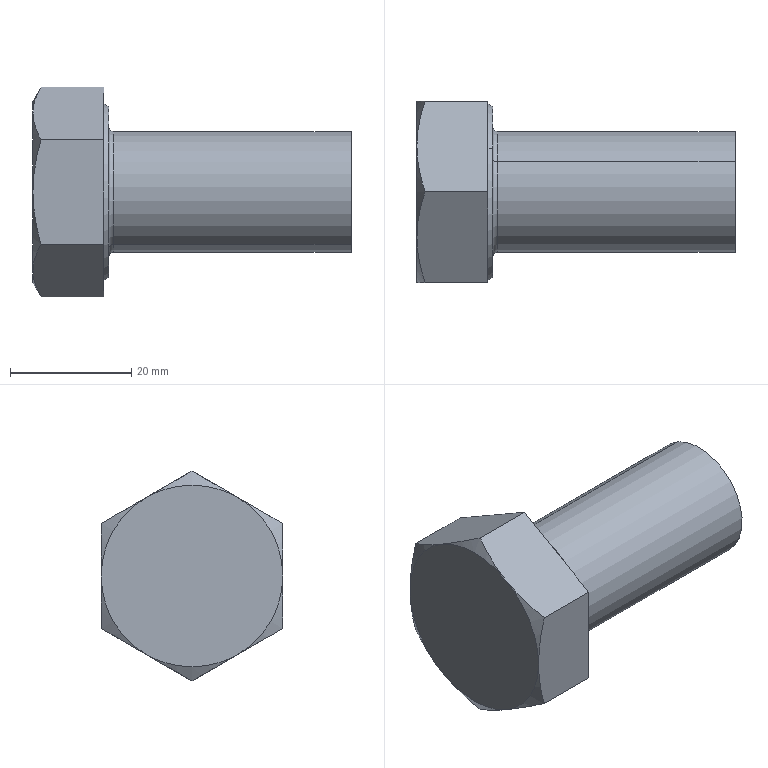Component | SolidWorks | GB_T5782-2016[HexHeadBoltM20_40]-1 | 1 solid | 22 faces | box 52.5 x 30 x 34.64 mm | volume 22181 mm3 | plane 10 | cone 8 | torus 2 | cylinder 2 | commonest cylinder face diameters 20 x2
build123d program:
from build123d import *

# Parameters (mm, degrees)
BASE_EXTRUDE_DEPTH = 12.5
FILLET_2_R         = 0.8
MOVE_FACE1_BY      = 40


with BuildPart() as part:
    # Sketch1 → Base-Extrude (new body)
    with BuildSketch(Plane(origin=(0, 0, 0), x_dir=(0, 0, -1), z_dir=(1, 0, 0))):
        Polygon((15, 8.66), (15, -8.66), (0, -17.321), (-15, -8.66), (-15, 8.66), (0, 17.321), align=None)
    extrude(amount=BASE_EXTRUDE_DEPTH)

    # Sketch2 → Revolve1 (revolve)
    with BuildSketch(Plane.XY, mode=Mode.PRIVATE) as revolve1_sk:
        Polygon((0, 0), (92.5, 0), (92.5, 7.835), (92.5, 10), (46.5, 10), (0, 10), align=None)
    revolve(revolve1_sk.sketch.rotate(Axis((0, 0, 0), (1, 0, 0)), 90), axis=Axis((0, 0, 0), (1, 0, 0)))

    # Sketch3 → Cut-Revolve1 (revolve, cut)
    with BuildSketch(Plane.XY):
        Polygon((0, 15), (4.226, 22.321), (4.226, 27.321), (-10, 27.321), (-10, 15), align=None)
    revolve(axis=Axis((0, 0, 0), (1, 0, 0)), mode=Mode.SUBTRACT)

    # Sketch4 → Cut-Revolve3 (revolve, cut)
    with BuildSketch(Plane.XY, mode=Mode.PRIVATE) as cut_revolve3_sk:
        Polygon((12.5, 14.095), (11.7, 14.557), (11.7, 17.321), (12.5, 17.321), align=None)
    revolve(cut_revolve3_sk.sketch.rotate(Axis((0, 0, 0), (1, 0, 0)), 90), axis=Axis((0, 0, 0), (1, 0, 0)), mode=Mode.SUBTRACT)

    # Fillet 2
    fillet_2_edges = [part.edges().sort_by_distance(p)[0] for p in [
        (12.5, 0, -10),
    ]]
    fillet(fillet_2_edges, radius=FILLET_2_R)

    # Move Face1: a face moved inward by 40.0
    extrude(part.faces().sort_by_distance((92.5, 0, 0))[0], amount=MOVE_FACE1_BY, dir=(-1, 0, 0), mode=Mode.SUBTRACT)


solid = part.part

# Placed as in the assembly
solid = solid.moved(Location((-212, -402, 70), (90, 0, 0)))
STEP:
#1=CARTESIAN_POINT('',(-7.823,-15.63,3.097));
#2=VERTEX_POINT('',#1);
#3=CARTESIAN_POINT('',(-7.823,-16.024,2.415));
#4=VERTEX_POINT('',#3);
#5=CARTESIAN_POINT('',(-7.823,-15.827,2.756));
#6=DIRECTION('',(1.,0.,0.));
#7=DIRECTION('',(0.,-0.5,-0.866));
#8=AXIS2_PLACEMENT_3D('',#5,#6,#7);
#9=CIRCLE('',#8,0.3937);
#10=EDGE_CURVE('',#2,#4,#9,.T.);
#11=ORIENTED_EDGE('',*,*,#10,.F.);
#12=CARTESIAN_POINT('',(-7.854,-15.614,3.124));
#13=VERTEX_POINT('',#12);
#14=CARTESIAN_POINT('',(-7.823,-15.614,3.124));
#15=DIRECTION('',(0.,0.866,-0.5));
#16=DIRECTION('',(0.,0.5,0.866));
#17=AXIS2_PLACEMENT_3D('',#14,#15,#16);
#18=CIRCLE('',#17,0.0315);
#19=EDGE_CURVE('',#2,#13,#18,.T.);
#20=ORIENTED_EDGE('',*,*,#19,.T.);
#21=CARTESIAN_POINT('',(-7.854,-16.039,2.388));
#22=VERTEX_POINT('',#21);
#23=CARTESIAN_POINT('',(-7.854,-15.827,2.756));
#24=DIRECTION('',(-1.,0.,0.));
#25=DIRECTION('',(0.,-0.5,-0.866));
#26=AXIS2_PLACEMENT_3D('',#23,#24,#25);
#27=CIRCLE('',#26,0.4252);
#28=EDGE_CURVE('',#22,#13,#27,.T.);
#29=ORIENTED_EDGE('',*,*,#28,.F.);
#30=CARTESIAN_POINT('',(-7.823,-16.039,2.388));
#31=DIRECTION('',(0.,-0.866,0.5));
#32=DIRECTION('',(0.,-0.5,-0.866));
#33=AXIS2_PLACEMENT_3D('',#30,#31,#32);
#34=CIRCLE('',#33,0.0315);
#35=EDGE_CURVE('',#4,#22,#34,.T.);
#36=ORIENTED_EDGE('',*,*,#35,.F.);
#37=EDGE_LOOP('',(#11,#20,#29,#36));
#38=FACE_OUTER_BOUND('',#37,.T.);
#39=CARTESIAN_POINT('',(-7.823,-15.827,2.756));
#40=DIRECTION('',(1.,0.,0.));
#41=DIRECTION('',(0.,-0.5,-0.866));
#42=AXIS2_PLACEMENT_3D('',#39,#40,#41);
#43=TOROIDAL_SURFACE('',#42,0.4252,0.0315);
#44=ADVANCED_FACE('',(#38),#43,.F.);
#45=CARTESIAN_POINT('',(-6.28,-15.63,3.097));
#46=VERTEX_POINT('',#45);
#47=CARTESIAN_POINT('',(-6.28,-16.024,2.415));
#48=VERTEX_POINT('',#47);
#49=CARTESIAN_POINT('',(-6.28,-15.827,2.756));
#50=DIRECTION('',(-1.,0.,0.));
#51=DIRECTION('',(0.,0.5,0.866));
#52=AXIS2_PLACEMENT_3D('',#49,#50,#51);
#53=CIRCLE('',#52,0.3937);
#54=EDGE_CURVE('',#46,#48,#53,.T.);
#55=ORIENTED_EDGE('',*,*,#54,.T.);
#56=CARTESIAN_POINT('',(-8.346,-16.024,2.415));
#57=DIRECTION('',(-1.,0.,0.));
#58=VECTOR('',#57,39.37);
#59=LINE('',#56,#58);
#60=EDGE_CURVE('',#48,#4,#59,.T.);
#61=ORIENTED_EDGE('',*,*,#60,.T.);
#62=CARTESIAN_POINT('',(-7.823,-15.827,2.756));
#63=DIRECTION('',(1.,0.,0.));
#64=DIRECTION('',(0.,-0.5,-0.866));
#65=AXIS2_PLACEMENT_3D('',#62,#63,#64);
#66=CIRCLE('',#65,0.3937);
#67=EDGE_CURVE('',#4,#2,#66,.T.);
#68=ORIENTED_EDGE('',*,*,#67,.T.);
#69=CARTESIAN_POINT('',(-8.346,-15.63,3.097));
#70=DIRECTION('',(-1.,0.,0.));
#71=VECTOR('',#70,39.37);
#72=LINE('',#69,#71);
#73=EDGE_CURVE('',#46,#2,#72,.T.);
#74=ORIENTED_EDGE('',*,*,#73,.F.);
#75=EDGE_LOOP('',(#55,#61,#68,#74));
#76=FACE_OUTER_BOUND('',#75,.T.);
#77=CARTESIAN_POINT('',(-8.346,-15.827,2.756));
#78=DIRECTION('',(-1.,0.,0.));
#79=DIRECTION('',(0.,0.5,0.866));
#80=AXIS2_PLACEMENT_3D('',#77,#78,#79);
#81=CYLINDRICAL_SURFACE('',#80,0.3937);
#82=ADVANCED_FACE('',(#76),#81,.T.);
#83=CARTESIAN_POINT('',(-7.854,-15.549,3.236));
#84=VERTEX_POINT('',#83);
#85=CARTESIAN_POINT('',(-7.854,-16.104,2.275));
#86=VERTEX_POINT('',#85);
#87=CARTESIAN_POINT('',(-7.854,-15.827,2.756));
#88=DIRECTION('',(-1.,0.,0.));
#89=DIRECTION('',(0.,0.5,0.866));
#90=AXIS2_PLACEMENT_3D('',#87,#88,#89);
#91=CIRCLE('',#90,0.5549);
#92=EDGE_CURVE('',#84,#86,#91,.T.);
#93=ORIENTED_EDGE('',*,*,#92,.T.);
#94=CARTESIAN_POINT('',(-7.886,-16.113,2.26));
#95=VERTEX_POINT('',#94);
#96=CARTESIAN_POINT('',(-7.886,-16.113,2.26));
#97=DIRECTION('',(-0.866,-0.25,-0.433));
#98=VECTOR('',#97,39.37);
#99=LINE('',#96,#98);
#100=EDGE_CURVE('',#86,#95,#99,.T.);
#101=ORIENTED_EDGE('',*,*,#100,.T.);
#102=CARTESIAN_POINT('',(-7.886,-15.54,3.252));
#103=VERTEX_POINT('',#102);
#104=CARTESIAN_POINT('',(-7.886,-15.827,2.756));
#105=DIRECTION('',(-1.,0.,0.));
#106=DIRECTION('',(0.,0.5,0.866));
#107=AXIS2_PLACEMENT_3D('',#104,#105,#106);
#108=CIRCLE('',#107,0.5731);
#109=EDGE_CURVE('',#103,#95,#108,.T.);
#110=ORIENTED_EDGE('',*,*,#109,.F.);
#111=CARTESIAN_POINT('',(-7.886,-15.54,3.252));
#112=DIRECTION('',(-0.866,0.25,0.433));
#113=VECTOR('',#112,39.37);
#114=LINE('',#111,#113);
#115=EDGE_CURVE('',#84,#103,#114,.T.);
#116=ORIENTED_EDGE('',*,*,#115,.F.);
#117=EDGE_LOOP('',(#93,#101,#110,#116));
#118=FACE_OUTER_BOUND('',#117,.T.);
#119=CARTESIAN_POINT('',(-7.886,-15.827,2.756));
#120=DIRECTION('',(-1.,0.,0.));
#121=DIRECTION('',(0.,0.5,0.866));
#122=AXIS2_PLACEMENT_3D('',#119,#120,#121);
#123=CONICAL_SURFACE('',#122,0.5731,0.5236);
#124=ADVANCED_FACE('',(#118),#123,.T.);
#125=CARTESIAN_POINT('',(-7.886,-15.827,2.074));
#126=VERTEX_POINT('',#125);
#127=CARTESIAN_POINT('',(-7.886,-15.236,2.415));
#128=VERTEX_POINT('',#127);
#129=CARTESIAN_POINT('',(-7.886,-15.827,2.074));
#130=DIRECTION('',(0.,0.866,0.5));
#131=VECTOR('',#130,39.37);
#132=LINE('',#129,#131);
#133=EDGE_CURVE('',#126,#128,#132,.T.);
#134=ORIENTED_EDGE('',*,*,#133,.F.);
#135=CARTESIAN_POINT('',(-8.294,-15.827,2.074));
#136=VERTEX_POINT('',#135);
#137=CARTESIAN_POINT('',(-7.854,-15.827,2.074));
#138=DIRECTION('',(-1.,0.,0.));
#139=VECTOR('',#138,39.37);
#140=LINE('',#137,#139);
#141=EDGE_CURVE('',#126,#136,#140,.T.);
#142=ORIENTED_EDGE('',*,*,#141,.T.);
#143=CARTESIAN_POINT('',(-8.346,-15.531,2.244));
#144=VERTEX_POINT('',#143);
#145=CARTESIAN_POINT('',(-8.346,-15.531,2.244));
#146=CARTESIAN_POINT('',(-8.346,-15.557,2.23));
#147=CARTESIAN_POINT('',(-8.345,-15.582,2.215));
#148=CARTESIAN_POINT('',(-8.34,-15.632,2.187));
#149=CARTESIAN_POINT('',(-8.337,-15.656,2.172));
#150=CARTESIAN_POINT('',(-8.323,-15.73,2.13));
#151=CARTESIAN_POINT('',(-8.31,-15.779,2.102));
#152=CARTESIAN_POINT('',(-8.294,-15.827,2.074));
#153=B_SPLINE_CURVE_WITH_KNOTS('',3,(#145,#146,#147,#148,#149,#150,#151,#152),.UNSPECIFIED.,.F.,.F.,(4,2,2,4),(0.008763,0.01095,0.01313,0.01749),.UNSPECIFIED.);
#154=EDGE_CURVE('',#144,#136,#153,.T.);
#155=ORIENTED_EDGE('',*,*,#154,.F.);
#156=CARTESIAN_POINT('',(-8.294,-15.236,2.415));
#157=VERTEX_POINT('',#156);
#158=CARTESIAN_POINT('',(-8.294,-15.236,2.415));
#159=CARTESIAN_POINT('',(-8.31,-15.285,2.387));
#160=CARTESIAN_POINT('',(-8.323,-15.333,2.359));
#161=CARTESIAN_POINT('',(-8.341,-15.432,2.302));
#162=CARTESIAN_POINT('',(-8.346,-15.481,2.274));
#163=CARTESIAN_POINT('',(-8.346,-15.531,2.244));
#164=B_SPLINE_CURVE_WITH_KNOTS('',3,(#158,#159,#160,#161,#162,#163),.UNSPECIFIED.,.F.,.F.,(4,2,4),(0.00000024,0.004382,0.008763),.UNSPECIFIED.);
#165=EDGE_CURVE('',#157,#144,#164,.T.);
#166=ORIENTED_EDGE('',*,*,#165,.F.);
#167=CARTESIAN_POINT('',(-7.854,-15.236,2.415));
#168=DIRECTION('',(-1.,0.,0.));
#169=VECTOR('',#168,39.37);
#170=LINE('',#167,#169);
#171=EDGE_CURVE('',#128,#157,#170,.T.);
#172=ORIENTED_EDGE('',*,*,#171,.F.);
#173=EDGE_LOOP('',(#134,#142,#155,#166,#172));
#174=FACE_OUTER_BOUND('',#173,.T.);
#175=CARTESIAN_POINT('',(-7.854,-15.827,2.074));
#176=DIRECTION('',(0.,-0.5,0.866));
#177=DIRECTION('',(0.,-0.866,-0.5));
#178=AXIS2_PLACEMENT_3D('',#175,#176,#177);
#179=PLANE('',#178);
#180=ADVANCED_FACE('',(#174),#179,.F.);
#181=CARTESIAN_POINT('',(-7.886,-15.236,3.097));
#182=VERTEX_POINT('',#181);
#183=CARTESIAN_POINT('',(-7.886,-15.236,2.415));
#184=DIRECTION('',(0.,-0.,1.));
#185=VECTOR('',#184,39.37);
#186=LINE('',#183,#185);
#187=EDGE_CURVE('',#128,#182,#186,.T.);
#188=ORIENTED_EDGE('',*,*,#187,.F.);
#189=ORIENTED_EDGE('',*,*,#171,.T.);
#190=CARTESIAN_POINT('',(-8.346,-15.236,2.756));
#191=VERTEX_POINT('',#190);
#192=CARTESIAN_POINT('',(-8.346,-15.236,2.756));
#193=CARTESIAN_POINT('',(-8.346,-15.236,2.727));
#194=CARTESIAN_POINT('',(-8.345,-15.236,2.698));
#195=CARTESIAN_POINT('',(-8.34,-15.236,2.64));
#196=CARTESIAN_POINT('',(-8.337,-15.236,2.612));
#197=CARTESIAN_POINT('',(-8.323,-15.236,2.527));
#198=CARTESIAN_POINT('',(-8.31,-15.236,2.471));
#199=CARTESIAN_POINT('',(-8.294,-15.236,2.415));
#200=B_SPLINE_CURVE_WITH_KNOTS('',3,(#192,#193,#194,#195,#196,#197,#198,#199),.UNSPECIFIED.,.F.,.F.,(4,2,2,4),(0.008763,0.01095,0.01313,0.01749),.UNSPECIFIED.);
#201=EDGE_CURVE('',#191,#157,#200,.T.);
#202=ORIENTED_EDGE('',*,*,#201,.F.);
#203=CARTESIAN_POINT('',(-8.294,-15.236,3.097));
#204=VERTEX_POINT('',#203);
#205=CARTESIAN_POINT('',(-8.294,-15.236,3.097));
#206=CARTESIAN_POINT('',(-8.31,-15.236,3.041));
#207=CARTESIAN_POINT('',(-8.323,-15.236,2.985));
#208=CARTESIAN_POINT('',(-8.341,-15.236,2.871));
#209=CARTESIAN_POINT('',(-8.346,-15.236,2.814));
#210=CARTESIAN_POINT('',(-8.346,-15.236,2.756));
#211=B_SPLINE_CURVE_WITH_KNOTS('',3,(#205,#206,#207,#208,#209,#210),.UNSPECIFIED.,.F.,.F.,(4,2,4),(0.00000024,0.004382,0.008763),.UNSPECIFIED.);
#212=EDGE_CURVE('',#204,#191,#211,.T.);
#213=ORIENTED_EDGE('',*,*,#212,.F.);
#214=CARTESIAN_POINT('',(-7.854,-15.236,3.097));
#215=DIRECTION('',(-1.,0.,0.));
#216=VECTOR('',#215,39.37);
#217=LINE('',#214,#216);
#218=EDGE_CURVE('',#182,#204,#217,.T.);
#219=ORIENTED_EDGE('',*,*,#218,.F.);
#220=EDGE_LOOP('',(#188,#189,#202,#213,#219));
#221=FACE_OUTER_BOUND('',#220,.T.);
#222=CARTESIAN_POINT('',(-7.854,-15.236,2.415));
#223=DIRECTION('',(0.,-1.,-0.));
#224=DIRECTION('',(0.,0.,-1.));
#225=AXIS2_PLACEMENT_3D('',#222,#223,#224);
#226=PLANE('',#225);
#227=ADVANCED_FACE('',(#221),#226,.F.);
#228=CARTESIAN_POINT('',(-7.886,-15.827,3.438));
#229=VERTEX_POINT('',#228);
#230=CARTESIAN_POINT('',(-7.886,-15.236,3.097));
#231=DIRECTION('',(0.,-0.866,0.5));
#232=VECTOR('',#231,39.37);
#233=LINE('',#230,#232);
#234=EDGE_CURVE('',#182,#229,#233,.T.);
#235=ORIENTED_EDGE('',*,*,#234,.F.);
#236=ORIENTED_EDGE('',*,*,#218,.T.);
#237=CARTESIAN_POINT('',(-8.346,-15.531,3.267));
#238=VERTEX_POINT('',#237);
#239=CARTESIAN_POINT('',(-8.346,-15.531,3.267));
#240=CARTESIAN_POINT('',(-8.346,-15.507,3.253));
#241=CARTESIAN_POINT('',(-8.345,-15.481,3.238));
#242=CARTESIAN_POINT('',(-8.34,-15.431,3.209));
#243=CARTESIAN_POINT('',(-8.337,-15.406,3.195));
#244=CARTESIAN_POINT('',(-8.323,-15.332,3.152));
#245=CARTESIAN_POINT('',(-8.31,-15.284,3.124));
#246=CARTESIAN_POINT('',(-8.294,-15.236,3.097));
#247=B_SPLINE_CURVE_WITH_KNOTS('',3,(#239,#240,#241,#242,#243,#244,#245,#246),.UNSPECIFIED.,.F.,.F.,(4,2,2,4),(0.02466,0.02686,0.02905,0.03344),.UNSPECIFIED.);
#248=EDGE_CURVE('',#238,#204,#247,.T.);
#249=ORIENTED_EDGE('',*,*,#248,.F.);
#250=CARTESIAN_POINT('',(-8.294,-15.827,3.438));
#251=VERTEX_POINT('',#250);
#252=CARTESIAN_POINT('',(-8.294,-15.827,3.438));
#253=CARTESIAN_POINT('',(-8.31,-15.779,3.41));
#254=CARTESIAN_POINT('',(-8.323,-15.73,3.382));
#255=CARTESIAN_POINT('',(-8.341,-15.631,3.325));
#256=CARTESIAN_POINT('',(-8.346,-15.581,3.296));
#257=CARTESIAN_POINT('',(-8.346,-15.531,3.267));
#258=B_SPLINE_CURVE_WITH_KNOTS('',3,(#252,#253,#254,#255,#256,#257),.UNSPECIFIED.,.F.,.F.,(4,2,4),(0.0159,0.02028,0.02466),.UNSPECIFIED.);
#259=EDGE_CURVE('',#251,#238,#258,.T.);
#260=ORIENTED_EDGE('',*,*,#259,.F.);
#261=CARTESIAN_POINT('',(-7.854,-15.827,3.438));
#262=DIRECTION('',(-1.,0.,0.));
#263=VECTOR('',#262,39.37);
#264=LINE('',#261,#263);
#265=EDGE_CURVE('',#229,#251,#264,.T.);
#266=ORIENTED_EDGE('',*,*,#265,.F.);
#267=EDGE_LOOP('',(#235,#236,#249,#260,#266));
#268=FACE_OUTER_BOUND('',#267,.T.);
#269=CARTESIAN_POINT('',(-7.854,-15.236,3.097));
#270=DIRECTION('',(0.,-0.5,-0.866));
#271=DIRECTION('',(-1.,0.,0.));
#272=AXIS2_PLACEMENT_3D('',#269,#270,#271);
#273=PLANE('',#272);
#274=ADVANCED_FACE('',(#268),#273,.F.);
#275=CARTESIAN_POINT('',(-7.886,-16.417,3.097));
#276=VERTEX_POINT('',#275);
#277=CARTESIAN_POINT('',(-7.886,-16.417,3.097));
#278=DIRECTION('',(0.,-0.866,-0.5));
#279=VECTOR('',#278,39.37);
#280=LINE('',#277,#279);
#281=EDGE_CURVE('',#229,#276,#280,.T.);
#282=ORIENTED_EDGE('',*,*,#281,.F.);
#283=ORIENTED_EDGE('',*,*,#265,.T.);
#284=CARTESIAN_POINT('',(-8.346,-16.122,3.267));
#285=VERTEX_POINT('',#284);
#286=CARTESIAN_POINT('',(-8.346,-16.122,3.267));
#287=CARTESIAN_POINT('',(-8.346,-16.097,3.282));
#288=CARTESIAN_POINT('',(-8.345,-16.072,3.296));
#289=CARTESIAN_POINT('',(-8.34,-16.022,3.325));
#290=CARTESIAN_POINT('',(-8.337,-15.997,3.339));
#291=CARTESIAN_POINT('',(-8.323,-15.924,3.382));
#292=CARTESIAN_POINT('',(-8.31,-15.875,3.41));
#293=CARTESIAN_POINT('',(-8.294,-15.827,3.438));
#294=B_SPLINE_CURVE_WITH_KNOTS('',3,(#286,#287,#288,#289,#290,#291,#292,#293),.UNSPECIFIED.,.F.,.F.,(4,2,2,4),(0.008763,0.01095,0.01313,0.01749),.UNSPECIFIED.);
#295=EDGE_CURVE('',#285,#251,#294,.T.);
#296=ORIENTED_EDGE('',*,*,#295,.F.);
#297=CARTESIAN_POINT('',(-8.294,-16.417,3.097));
#298=VERTEX_POINT('',#297);
#299=CARTESIAN_POINT('',(-8.294,-16.417,3.097));
#300=CARTESIAN_POINT('',(-8.31,-16.369,3.125));
#301=CARTESIAN_POINT('',(-8.323,-16.32,3.153));
#302=CARTESIAN_POINT('',(-8.341,-16.222,3.21));
#303=CARTESIAN_POINT('',(-8.346,-16.172,3.238));
#304=CARTESIAN_POINT('',(-8.346,-16.122,3.267));
#305=B_SPLINE_CURVE_WITH_KNOTS('',3,(#299,#300,#301,#302,#303,#304),.UNSPECIFIED.,.F.,.F.,(4,2,4),(0.00000024,0.004382,0.008763),.UNSPECIFIED.);
#306=EDGE_CURVE('',#298,#285,#305,.T.);
#307=ORIENTED_EDGE('',*,*,#306,.F.);
#308=CARTESIAN_POINT('',(-7.854,-16.417,3.097));
#309=DIRECTION('',(-1.,0.,0.));
#310=VECTOR('',#309,39.37);
#311=LINE('',#308,#310);
#312=EDGE_CURVE('',#276,#298,#311,.T.);
#313=ORIENTED_EDGE('',*,*,#312,.F.);
#314=EDGE_LOOP('',(#282,#283,#296,#307,#313));
#315=FACE_OUTER_BOUND('',#314,.T.);
#316=CARTESIAN_POINT('',(-7.854,-16.417,3.097));
#317=DIRECTION('',(0.,0.5,-0.866));
#318=DIRECTION('',(0.,0.866,0.5));
#319=AXIS2_PLACEMENT_3D('',#316,#317,#318);
#320=PLANE('',#319);
#321=ADVANCED_FACE('',(#315),#320,.F.);
#322=CARTESIAN_POINT('',(-7.886,-16.417,2.415));
#323=VERTEX_POINT('',#322);
#324=CARTESIAN_POINT('',(-7.886,-16.417,2.415));
#325=DIRECTION('',(0.,0.,-1.));
#326=VECTOR('',#325,39.37);
#327=LINE('',#324,#326);
#328=EDGE_CURVE('',#276,#323,#327,.T.);
#329=ORIENTED_EDGE('',*,*,#328,.F.);
#330=ORIENTED_EDGE('',*,*,#312,.T.);
#331=CARTESIAN_POINT('',(-8.346,-16.417,2.756));
#332=VERTEX_POINT('',#331);
#333=CARTESIAN_POINT('',(-8.346,-16.417,2.756));
#334=CARTESIAN_POINT('',(-8.346,-16.417,2.785));
#335=CARTESIAN_POINT('',(-8.345,-16.417,2.814));
#336=CARTESIAN_POINT('',(-8.34,-16.417,2.871));
#337=CARTESIAN_POINT('',(-8.337,-16.417,2.9));
#338=CARTESIAN_POINT('',(-8.323,-16.417,2.985));
#339=CARTESIAN_POINT('',(-8.31,-16.417,3.041));
#340=CARTESIAN_POINT('',(-8.294,-16.417,3.097));
#341=B_SPLINE_CURVE_WITH_KNOTS('',3,(#333,#334,#335,#336,#337,#338,#339,#340),.UNSPECIFIED.,.F.,.F.,(4,2,2,4),(0.008763,0.01095,0.01313,0.01749),.UNSPECIFIED.);
#342=EDGE_CURVE('',#332,#298,#341,.T.);
#343=ORIENTED_EDGE('',*,*,#342,.F.);
#344=CARTESIAN_POINT('',(-8.294,-16.417,2.415));
#345=VERTEX_POINT('',#344);
#346=CARTESIAN_POINT('',(-8.294,-16.417,2.415));
#347=CARTESIAN_POINT('',(-8.31,-16.417,2.471));
#348=CARTESIAN_POINT('',(-8.323,-16.417,2.527));
#349=CARTESIAN_POINT('',(-8.341,-16.417,2.64));
#350=CARTESIAN_POINT('',(-8.346,-16.417,2.698));
#351=CARTESIAN_POINT('',(-8.346,-16.417,2.756));
#352=B_SPLINE_CURVE_WITH_KNOTS('',3,(#346,#347,#348,#349,#350,#351),.UNSPECIFIED.,.F.,.F.,(4,2,4),(0.00000024,0.004382,0.008763),.UNSPECIFIED.);
#353=EDGE_CURVE('',#345,#332,#352,.T.);
#354=ORIENTED_EDGE('',*,*,#353,.F.);
#355=CARTESIAN_POINT('',(-7.854,-16.417,2.415));
#356=DIRECTION('',(-1.,0.,0.));
#357=VECTOR('',#356,39.37);
#358=LINE('',#355,#357);
#359=EDGE_CURVE('',#323,#345,#358,.T.);
#360=ORIENTED_EDGE('',*,*,#359,.F.);
#361=EDGE_LOOP('',(#329,#330,#343,#354,#360));
#362=FACE_OUTER_BOUND('',#361,.T.);
#363=CARTESIAN_POINT('',(-7.854,-16.417,2.415));
#364=DIRECTION('',(0.,1.,0.));
#365=DIRECTION('',(0.,-0.,1.));
#366=AXIS2_PLACEMENT_3D('',#363,#364,#365);
#367=PLANE('',#366);
#368=ADVANCED_FACE('',(#362),#367,.F.);
#369=CARTESIAN_POINT('',(-7.886,-15.827,2.074));
#370=DIRECTION('',(0.,0.866,-0.5));
#371=VECTOR('',#370,39.37);
#372=LINE('',#369,#371);
#373=EDGE_CURVE('',#323,#126,#372,.T.);
#374=ORIENTED_EDGE('',*,*,#373,.F.);
#375=ORIENTED_EDGE('',*,*,#359,.T.);
#376=CARTESIAN_POINT('',(-8.346,-16.122,2.244));
#377=VERTEX_POINT('',#376);
#378=CARTESIAN_POINT('',(-8.346,-16.122,2.244));
#379=CARTESIAN_POINT('',(-8.346,-16.172,2.273));
#380=CARTESIAN_POINT('',(-8.341,-16.222,2.302));
#381=CARTESIAN_POINT('',(-8.323,-16.32,2.359));
#382=CARTESIAN_POINT('',(-8.31,-16.369,2.387));
#383=CARTESIAN_POINT('',(-8.294,-16.417,2.415));
#384=B_SPLINE_CURVE_WITH_KNOTS('',3,(#378,#379,#380,#381,#382,#383),.UNSPECIFIED.,.F.,.F.,(4,2,4),(0.04846,0.05285,0.05723),.UNSPECIFIED.);
#385=EDGE_CURVE('',#377,#345,#384,.T.);
#386=ORIENTED_EDGE('',*,*,#385,.F.);
#387=CARTESIAN_POINT('',(-8.294,-15.827,2.074));
#388=CARTESIAN_POINT('',(-8.31,-15.875,2.102));
#389=CARTESIAN_POINT('',(-8.323,-15.923,2.129));
#390=CARTESIAN_POINT('',(-8.337,-15.997,2.172));
#391=CARTESIAN_POINT('',(-8.34,-16.022,2.187));
#392=CARTESIAN_POINT('',(-8.345,-16.072,2.216));
#393=CARTESIAN_POINT('',(-8.346,-16.097,2.23));
#394=CARTESIAN_POINT('',(-8.346,-16.122,2.244));
#395=B_SPLINE_CURVE_WITH_KNOTS('',3,(#387,#388,#389,#390,#391,#392,#393,#394),.UNSPECIFIED.,.F.,.F.,(4,2,2,4),(0.03969,0.04407,0.04627,0.04846),.UNSPECIFIED.);
#396=EDGE_CURVE('',#136,#377,#395,.T.);
#397=ORIENTED_EDGE('',*,*,#396,.F.);
#398=ORIENTED_EDGE('',*,*,#141,.F.);
#399=EDGE_LOOP('',(#374,#375,#386,#397,#398));
#400=FACE_OUTER_BOUND('',#399,.T.);
#401=CARTESIAN_POINT('',(-7.854,-15.827,2.074));
#402=DIRECTION('',(0.,0.5,0.866));
#403=DIRECTION('',(0.,-0.866,0.5));
#404=AXIS2_PLACEMENT_3D('',#401,#402,#403);
#405=PLANE('',#404);
#406=ADVANCED_FACE('',(#400),#405,.F.);
#407=ORIENTED_EDGE('',*,*,#353,.T.);
#408=CARTESIAN_POINT('',(-8.346,-15.827,2.756));
#409=DIRECTION('',(1.,0.,0.));
#410=DIRECTION('',(0.,-0.5,-0.866));
#411=AXIS2_PLACEMENT_3D('',#408,#409,#410);
#412=CIRCLE('',#411,0.5906);
#413=EDGE_CURVE('',#332,#377,#412,.T.);
#414=ORIENTED_EDGE('',*,*,#413,.T.);
#415=ORIENTED_EDGE('',*,*,#385,.T.);
#416=EDGE_LOOP('',(#407,#414,#415));
#417=FACE_OUTER_BOUND('',#416,.T.);
#418=CARTESIAN_POINT('',(-8.346,-15.827,2.756));
#419=DIRECTION('',(1.,0.,0.));
#420=DIRECTION('',(0.,-0.5,-0.866));
#421=AXIS2_PLACEMENT_3D('',#418,#419,#420);
#422=CONICAL_SURFACE('',#421,0.5906,1.047);
#423=ADVANCED_FACE('',(#417),#422,.T.);
#424=ORIENTED_EDGE('',*,*,#306,.T.);
#425=CARTESIAN_POINT('',(-8.346,-15.827,2.756));
#426=DIRECTION('',(1.,0.,0.));
#427=DIRECTION('',(0.,-0.5,-0.866));
#428=AXIS2_PLACEMENT_3D('',#425,#426,#427);
#429=CIRCLE('',#428,0.5906);
#430=EDGE_CURVE('',#285,#332,#429,.T.);
#431=ORIENTED_EDGE('',*,*,#430,.T.);
#432=ORIENTED_EDGE('',*,*,#342,.T.);
#433=EDGE_LOOP('',(#424,#431,#432));
#434=FACE_OUTER_BOUND('',#433,.T.);
#435=CARTESIAN_POINT('',(-8.346,-15.827,2.756));
#436=DIRECTION('',(1.,0.,0.));
#437=DIRECTION('',(0.,-0.5,-0.866));
#438=AXIS2_PLACEMENT_3D('',#435,#436,#437);
#439=CONICAL_SURFACE('',#438,0.5906,1.047);
#440=ADVANCED_FACE('',(#434),#439,.T.);
#441=ORIENTED_EDGE('',*,*,#259,.T.);
#442=CARTESIAN_POINT('',(-8.346,-15.827,2.756));
#443=DIRECTION('',(1.,0.,0.));
#444=DIRECTION('',(0.,-0.5,-0.866));
#445=AXIS2_PLACEMENT_3D('',#442,#443,#444);
#446=CIRCLE('',#445,0.5906);
#447=EDGE_CURVE('',#238,#285,#446,.T.);
#448=ORIENTED_EDGE('',*,*,#447,.T.);
#449=ORIENTED_EDGE('',*,*,#295,.T.);
#450=EDGE_LOOP('',(#441,#448,#449));
#451=FACE_OUTER_BOUND('',#450,.T.);
#452=CARTESIAN_POINT('',(-8.346,-15.827,2.756));
#453=DIRECTION('',(1.,0.,0.));
#454=DIRECTION('',(0.,-0.5,-0.866));
#455=AXIS2_PLACEMENT_3D('',#452,#453,#454);
#456=CONICAL_SURFACE('',#455,0.5906,1.047);
#457=ADVANCED_FACE('',(#451),#456,.T.);
#458=ORIENTED_EDGE('',*,*,#248,.T.);
#459=ORIENTED_EDGE('',*,*,#212,.T.);
#460=CARTESIAN_POINT('',(-8.346,-15.827,2.756));
#461=DIRECTION('',(-1.,0.,0.));
#462=DIRECTION('',(0.,0.5,0.866));
#463=AXIS2_PLACEMENT_3D('',#460,#461,#462);
#464=CIRCLE('',#463,0.5906);
#465=EDGE_CURVE('',#238,#191,#464,.T.);
#466=ORIENTED_EDGE('',*,*,#465,.F.);
#467=EDGE_LOOP('',(#458,#459,#466));
#468=FACE_OUTER_BOUND('',#467,.T.);
#469=CARTESIAN_POINT('',(-8.346,-15.827,2.756));
#470=DIRECTION('',(1.,0.,0.));
#471=DIRECTION('',(0.,-0.5,-0.866));
#472=AXIS2_PLACEMENT_3D('',#469,#470,#471);
#473=CONICAL_SURFACE('',#472,0.5906,1.047);
#474=ADVANCED_FACE('',(#468),#473,.T.);
#475=ORIENTED_EDGE('',*,*,#201,.T.);
#476=ORIENTED_EDGE('',*,*,#165,.T.);
#477=CARTESIAN_POINT('',(-8.346,-15.827,2.756));
#478=DIRECTION('',(1.,0.,0.));
#479=DIRECTION('',(0.,-0.5,-0.866));
#480=AXIS2_PLACEMENT_3D('',#477,#478,#479);
#481=CIRCLE('',#480,0.5906);
#482=EDGE_CURVE('',#144,#191,#481,.T.);
#483=ORIENTED_EDGE('',*,*,#482,.T.);
#484=EDGE_LOOP('',(#475,#476,#483));
#485=FACE_OUTER_BOUND('',#484,.T.);
#486=CARTESIAN_POINT('',(-8.346,-15.827,2.756));
#487=DIRECTION('',(1.,0.,0.));
#488=DIRECTION('',(0.,-0.5,-0.866));
#489=AXIS2_PLACEMENT_3D('',#486,#487,#488);
#490=CONICAL_SURFACE('',#489,0.5906,1.047);
#491=ADVANCED_FACE('',(#485),#490,.T.);
#492=ORIENTED_EDGE('',*,*,#154,.T.);
#493=ORIENTED_EDGE('',*,*,#396,.T.);
#494=CARTESIAN_POINT('',(-8.346,-15.827,2.756));
#495=DIRECTION('',(1.,0.,0.));
#496=DIRECTION('',(0.,-0.5,-0.866));
#497=AXIS2_PLACEMENT_3D('',#494,#495,#496);
#498=CIRCLE('',#497,0.5906);
#499=EDGE_CURVE('',#377,#144,#498,.T.);
#500=ORIENTED_EDGE('',*,*,#499,.T.);
#501=EDGE_LOOP('',(#492,#493,#500));
#502=FACE_OUTER_BOUND('',#501,.T.);
#503=CARTESIAN_POINT('',(-8.346,-15.827,2.756));
#504=DIRECTION('',(1.,0.,0.));
#505=DIRECTION('',(0.,-0.5,-0.866));
#506=AXIS2_PLACEMENT_3D('',#503,#504,#505);
#507=CONICAL_SURFACE('',#506,0.5906,1.047);
#508=ADVANCED_FACE('',(#502),#507,.T.);
#509=ORIENTED_EDGE('',*,*,#499,.F.);
#510=ORIENTED_EDGE('',*,*,#413,.F.);
#511=ORIENTED_EDGE('',*,*,#430,.F.);
#512=ORIENTED_EDGE('',*,*,#447,.F.);
#513=ORIENTED_EDGE('',*,*,#465,.T.);
#514=ORIENTED_EDGE('',*,*,#482,.F.);
#515=EDGE_LOOP('',(#509,#510,#511,#512,#513,#514));
#516=FACE_OUTER_BOUND('',#515,.T.);
#517=CARTESIAN_POINT('',(-8.346,-15.236,2.415));
#518=DIRECTION('',(1.,0.,0.));
#519=DIRECTION('',(0.,-0.5,-0.866));
#520=AXIS2_PLACEMENT_3D('',#517,#518,#519);
#521=PLANE('',#520);
#522=ADVANCED_FACE('',(#516),#521,.F.);
#523=ORIENTED_EDGE('',*,*,#109,.T.);
#524=CARTESIAN_POINT('',(-7.886,-15.827,2.756));
#525=DIRECTION('',(-1.,0.,0.));
#526=DIRECTION('',(0.,0.5,0.866));
#527=AXIS2_PLACEMENT_3D('',#524,#525,#526);
#528=CIRCLE('',#527,0.5731);
#529=EDGE_CURVE('',#95,#103,#528,.T.);
#530=ORIENTED_EDGE('',*,*,#529,.T.);
#531=EDGE_LOOP('',(#523,#530));
#532=FACE_BOUND('',#531,.T.);
#533=ORIENTED_EDGE('',*,*,#133,.T.);
#534=ORIENTED_EDGE('',*,*,#187,.T.);
#535=ORIENTED_EDGE('',*,*,#234,.T.);
#536=ORIENTED_EDGE('',*,*,#281,.T.);
#537=ORIENTED_EDGE('',*,*,#328,.T.);
#538=ORIENTED_EDGE('',*,*,#373,.T.);
#539=EDGE_LOOP('',(#533,#534,#535,#536,#537,#538));
#540=FACE_OUTER_BOUND('',#539,.T.);
#541=CARTESIAN_POINT('',(-7.886,-15.33,2.469));
#542=DIRECTION('',(1.,0.,0.));
#543=DIRECTION('',(0.,-0.5,-0.866));
#544=AXIS2_PLACEMENT_3D('',#541,#542,#543);
#545=PLANE('',#544);
#546=ADVANCED_FACE('',(#532,#540),#545,.T.);
#547=ORIENTED_EDGE('',*,*,#100,.F.);
#548=CARTESIAN_POINT('',(-7.854,-15.827,2.756));
#549=DIRECTION('',(-1.,0.,0.));
#550=DIRECTION('',(0.,0.5,0.866));
#551=AXIS2_PLACEMENT_3D('',#548,#549,#550);
#552=CIRCLE('',#551,0.5549);
#553=EDGE_CURVE('',#86,#84,#552,.T.);
#554=ORIENTED_EDGE('',*,*,#553,.T.);
#555=ORIENTED_EDGE('',*,*,#115,.T.);
#556=ORIENTED_EDGE('',*,*,#529,.F.);
#557=EDGE_LOOP('',(#547,#554,#555,#556));
#558=FACE_OUTER_BOUND('',#557,.T.);
#559=CARTESIAN_POINT('',(-7.886,-15.827,2.756));
#560=DIRECTION('',(-1.,0.,0.));
#561=DIRECTION('',(0.,0.5,0.866));
#562=AXIS2_PLACEMENT_3D('',#559,#560,#561);
#563=CONICAL_SURFACE('',#562,0.5731,0.5236);
#564=ADVANCED_FACE('',(#558),#563,.T.);
#565=ORIENTED_EDGE('',*,*,#54,.F.);
#566=CARTESIAN_POINT('',(-6.28,-15.827,2.756));
#567=DIRECTION('',(-1.,0.,0.));
#568=DIRECTION('',(0.,0.5,0.866));
#569=AXIS2_PLACEMENT_3D('',#566,#567,#568);
#570=CIRCLE('',#569,0.3937);
#571=EDGE_CURVE('',#48,#46,#570,.T.);
#572=ORIENTED_EDGE('',*,*,#571,.F.);
#573=EDGE_LOOP('',(#565,#572));
#574=FACE_OUTER_BOUND('',#573,.T.);
#575=CARTESIAN_POINT('',(-6.28,-15.827,2.756));
#576=DIRECTION('',(-1.,0.,0.));
#577=DIRECTION('',(0.,0.5,0.866));
#578=AXIS2_PLACEMENT_3D('',#575,#576,#577);
#579=PLANE('',#578);
#580=ADVANCED_FACE('',(#574),#579,.F.);
#581=ORIENTED_EDGE('',*,*,#60,.F.);
#582=ORIENTED_EDGE('',*,*,#571,.T.);
#583=ORIENTED_EDGE('',*,*,#73,.T.);
#584=ORIENTED_EDGE('',*,*,#10,.T.);
#585=EDGE_LOOP('',(#581,#582,#583,#584));
#586=FACE_OUTER_BOUND('',#585,.T.);
#587=CARTESIAN_POINT('',(-8.346,-15.827,2.756));
#588=DIRECTION('',(-1.,0.,0.));
#589=DIRECTION('',(0.,0.5,0.866));
#590=AXIS2_PLACEMENT_3D('',#587,#588,#589);
#591=CYLINDRICAL_SURFACE('',#590,0.3937);
#592=ADVANCED_FACE('',(#586),#591,.T.);
#593=ORIENTED_EDGE('',*,*,#28,.T.);
#594=CARTESIAN_POINT('',(-7.854,-15.827,2.756));
#595=DIRECTION('',(-1.,0.,0.));
#596=DIRECTION('',(0.,-0.5,-0.866));
#597=AXIS2_PLACEMENT_3D('',#594,#595,#596);
#598=CIRCLE('',#597,0.4252);
#599=EDGE_CURVE('',#13,#22,#598,.T.);
#600=ORIENTED_EDGE('',*,*,#599,.T.);
#601=EDGE_LOOP('',(#593,#600));
#602=FACE_BOUND('',#601,.T.);
#603=ORIENTED_EDGE('',*,*,#92,.F.);
#604=ORIENTED_EDGE('',*,*,#553,.F.);
#605=EDGE_LOOP('',(#603,#604));
#606=FACE_OUTER_BOUND('',#605,.T.);
#607=CARTESIAN_POINT('',(-7.854,-15.236,2.415));
#608=DIRECTION('',(1.,0.,0.));
#609=DIRECTION('',(0.,-0.5,-0.866));
#610=AXIS2_PLACEMENT_3D('',#607,#608,#609);
#611=PLANE('',#610);
#612=ADVANCED_FACE('',(#602,#606),#611,.T.);
#613=ORIENTED_EDGE('',*,*,#19,.F.);
#614=ORIENTED_EDGE('',*,*,#67,.F.);
#615=ORIENTED_EDGE('',*,*,#35,.T.);
#616=ORIENTED_EDGE('',*,*,#599,.F.);
#617=EDGE_LOOP('',(#613,#614,#615,#616));
#618=FACE_OUTER_BOUND('',#617,.T.);
#619=CARTESIAN_POINT('',(-7.823,-15.827,2.756));
#620=DIRECTION('',(1.,0.,0.));
#621=DIRECTION('',(0.,-0.5,-0.866));
#622=AXIS2_PLACEMENT_3D('',#619,#620,#621);
#623=TOROIDAL_SURFACE('',#622,0.4252,0.0315);
#624=ADVANCED_FACE('',(#618),#623,.F.);
#625=CLOSED_SHELL('',(#44,#82,#124,#180,#227,#274,#321,#368,#406,#423,#440,#457,#474,#491,#508,#522,#546,#564,#580,#592,#612,#624));
#626=MANIFOLD_SOLID_BREP('',#625);
#627=CARTESIAN_POINT('',(0.,0.,0.));
#628=DIRECTION('',(0.,0.,1.));
#629=DIRECTION('',(1.,0.,0.));
#630=AXIS2_PLACEMENT_3D('',#627,#628,#629);
#631=(LENGTH_UNIT()NAMED_UNIT(*)SI_UNIT($,.METRE.));
#632=LENGTH_MEASURE_WITH_UNIT(LENGTH_MEASURE(0.0254),#631);
#633=DIMENSIONAL_EXPONENTS(1.,0.,0.,0.,0.,0.,0.);
#634=(CONVERSION_BASED_UNIT('',#632)LENGTH_UNIT()NAMED_UNIT(#633));
#635=UNCERTAINTY_MEASURE_WITH_UNIT(LENGTH_MEASURE(0.00001),#634,'','');
#636=(NAMED_UNIT(*)PLANE_ANGLE_UNIT()SI_UNIT($,.RADIAN.));
#637=(NAMED_UNIT(*)SI_UNIT($,.STERADIAN.)SOLID_ANGLE_UNIT());
#638=(GEOMETRIC_REPRESENTATION_CONTEXT(3)GLOBAL_UNCERTAINTY_ASSIGNED_CONTEXT((#635))GLOBAL_UNIT_ASSIGNED_CONTEXT((#634,#636,#637))REPRESENTATION_CONTEXT('',''));
#639=ADVANCED_BREP_SHAPE_REPRESENTATION('',(#626,#630),#638);
#640=COLOUR_RGB('',0.7922,0.8196,0.9333);
#641=FILL_AREA_STYLE_COLOUR('',#640);
#642=FILL_AREA_STYLE('',(#641));
#643=SURFACE_STYLE_FILL_AREA(#642);
#644=SURFACE_SIDE_STYLE('',(#643));
#645=SURFACE_STYLE_USAGE(.BOTH.,#644);
#646=PRESENTATION_STYLE_ASSIGNMENT((#645));
#647=STYLED_ITEM('',(#646),#626);
#648=(LENGTH_UNIT()NAMED_UNIT(*)SI_UNIT($,.METRE.));
#649=LENGTH_MEASURE_WITH_UNIT(LENGTH_MEASURE(0.0254),#648);
#650=DIMENSIONAL_EXPONENTS(1.,0.,0.,0.,0.,0.,0.);
#651=(CONVERSION_BASED_UNIT('',#649)LENGTH_UNIT()NAMED_UNIT(#650));
#652=UNCERTAINTY_MEASURE_WITH_UNIT(LENGTH_MEASURE(0.00001),#651,'','');
#653=(NAMED_UNIT(*)PLANE_ANGLE_UNIT()SI_UNIT($,.RADIAN.));
#654=(NAMED_UNIT(*)SI_UNIT($,.STERADIAN.)SOLID_ANGLE_UNIT());
#655=(GEOMETRIC_REPRESENTATION_CONTEXT(3)GLOBAL_UNCERTAINTY_ASSIGNED_CONTEXT((#652))GLOBAL_UNIT_ASSIGNED_CONTEXT((#651,#653,#654))REPRESENTATION_CONTEXT('',''));
#656=MECHANICAL_DESIGN_GEOMETRIC_PRESENTATION_REPRESENTATION('',(#647),#655);
#657=PRESENTATION_LAYER_ASSIGNMENT('','',(#647));